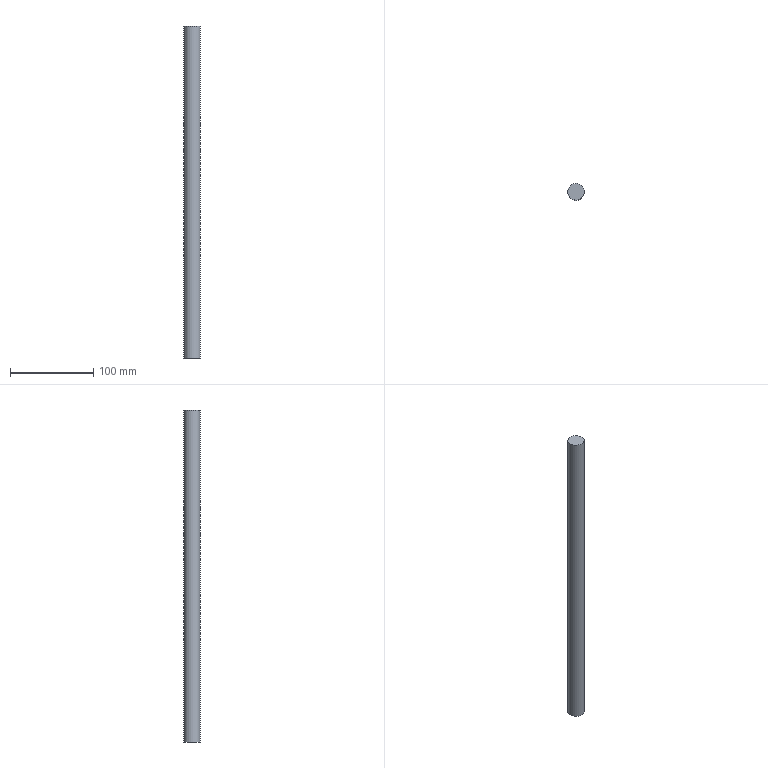Component | NX | D_2 | 1 solid | 3 faces | box 20 x 20 x 400 mm | volume 125664 mm3 | plane 2 | cylinder 1 | commonest cylinder face diameters 20 x1
STEP:
#1=CARTESIAN_POINT('',(0.,0.,0.));
#2=DIRECTION('',(0.,0.,1.));
#3=DIRECTION('',(1.,0.,0.));
#4=AXIS2_PLACEMENT_3D('',#1,#2,#3);
#5=CARTESIAN_POINT('',(850.763,-18.9,-161.891));
#6=VERTEX_POINT('',#5);
#7=CARTESIAN_POINT('',(860.,-15.069,-161.891));
#8=DIRECTION('',(0.,0.,-1.));
#9=DIRECTION('',(-0.9237,-0.383,0.));
#10=AXIS2_PLACEMENT_3D('',#7,#8,#9);
#11=CIRCLE('',#10,10.);
#12=CARTESIAN_POINT('',(860.,-15.069,-161.891));
#13=DIRECTION('',(0.,0.,1.));
#14=DIRECTION('',(0.9237,0.383,0.));
#15=AXIS2_PLACEMENT_3D('',#12,#13,#14);
#16=CYLINDRICAL_SURFACE('',#15,10.);
#17=CARTESIAN_POINT('',(9.425,0.));
#18=DIRECTION('',(-1.,0.));
#19=VECTOR('',#18,1.);
#20=LINE('',#17,#19);
#21=(GEOMETRIC_REPRESENTATION_CONTEXT(2)PARAMETRIC_REPRESENTATION_CONTEXT()REPRESENTATION_CONTEXT('',''));
#22=DEFINITIONAL_REPRESENTATION('',(#20),#21);
#23=PCURVE('',#16,#22);
#24=CARTESIAN_POINT('',(860.,-15.069,-161.891));
#25=DIRECTION('',(0.,0.,-1.));
#26=DIRECTION('',(-0.9237,-0.383,0.));
#27=AXIS2_PLACEMENT_3D('',#24,#25,#26);
#28=PLANE('',#27);
#29=CARTESIAN_POINT('',(0.,0.));
#30=DIRECTION('',(1.,0.));
#31=AXIS2_PLACEMENT_2D('',#29,#30);
#32=CIRCLE('',#31,10.);
#33=(GEOMETRIC_REPRESENTATION_CONTEXT(2)PARAMETRIC_REPRESENTATION_CONTEXT()REPRESENTATION_CONTEXT('',''));
#34=DEFINITIONAL_REPRESENTATION('',(#32),#33);
#35=PCURVE('',#28,#34);
#36=SURFACE_CURVE('',#11,(#23,#35),.PCURVE_S1.);
#37=EDGE_CURVE('',#6,#6,#36,.T.);
#38=ORIENTED_EDGE('',*,*,#37,.F.);
#39=CARTESIAN_POINT('',(850.763,-18.9,238.109));
#40=VERTEX_POINT('',#39);
#41=CARTESIAN_POINT('',(850.763,-18.9,-161.891));
#42=CARTESIAN_POINT('',(850.763,-18.9,238.109));
#43=B_SPLINE_CURVE_WITH_KNOTS('',1,(#41,#42),.UNSPECIFIED.,.F.,.F.,(2,2),(0.,400.),.PIECEWISE_BEZIER_KNOTS.);
#44=CARTESIAN_POINT('',(9.425,0.));
#45=DIRECTION('',(0.,1.));
#46=VECTOR('',#45,1.);
#47=LINE('',#44,#46);
#48=(GEOMETRIC_REPRESENTATION_CONTEXT(2)PARAMETRIC_REPRESENTATION_CONTEXT()REPRESENTATION_CONTEXT('',''));
#49=DEFINITIONAL_REPRESENTATION('',(#47),#48);
#50=PCURVE('',#16,#49);
#51=CARTESIAN_POINT('',(3.142,0.));
#52=DIRECTION('',(0.,1.));
#53=VECTOR('',#52,1.);
#54=LINE('',#51,#53);
#55=(GEOMETRIC_REPRESENTATION_CONTEXT(2)PARAMETRIC_REPRESENTATION_CONTEXT()REPRESENTATION_CONTEXT('',''));
#56=DEFINITIONAL_REPRESENTATION('',(#54),#55);
#57=PCURVE('',#16,#56);
#58=SEAM_CURVE('',#43,(#50,#57),.PCURVE_S1.);
#59=EDGE_CURVE('',#6,#40,#58,.T.);
#60=ORIENTED_EDGE('',*,*,#59,.T.);
#61=CARTESIAN_POINT('',(860.,-15.069,238.109));
#62=DIRECTION('',(0.,0.,-1.));
#63=DIRECTION('',(-0.9237,-0.383,0.));
#64=AXIS2_PLACEMENT_3D('',#61,#62,#63);
#65=CIRCLE('',#64,10.);
#66=CARTESIAN_POINT('',(9.425,400.));
#67=DIRECTION('',(-1.,0.));
#68=VECTOR('',#67,1.);
#69=LINE('',#66,#68);
#70=(GEOMETRIC_REPRESENTATION_CONTEXT(2)PARAMETRIC_REPRESENTATION_CONTEXT()REPRESENTATION_CONTEXT('',''));
#71=DEFINITIONAL_REPRESENTATION('',(#69),#70);
#72=PCURVE('',#16,#71);
#73=CARTESIAN_POINT('',(860.,-15.069,238.109));
#74=DIRECTION('',(0.,0.,-1.));
#75=DIRECTION('',(-0.9237,-0.383,0.));
#76=AXIS2_PLACEMENT_3D('',#73,#74,#75);
#77=PLANE('',#76);
#78=CARTESIAN_POINT('',(0.,0.));
#79=DIRECTION('',(1.,0.));
#80=AXIS2_PLACEMENT_2D('',#78,#79);
#81=CIRCLE('',#80,10.);
#82=(GEOMETRIC_REPRESENTATION_CONTEXT(2)PARAMETRIC_REPRESENTATION_CONTEXT()REPRESENTATION_CONTEXT('',''));
#83=DEFINITIONAL_REPRESENTATION('',(#81),#82);
#84=PCURVE('',#77,#83);
#85=SURFACE_CURVE('',#65,(#72,#84),.PCURVE_S1.);
#86=EDGE_CURVE('',#40,#40,#85,.T.);
#87=ORIENTED_EDGE('',*,*,#86,.T.);
#88=ORIENTED_EDGE('',*,*,#59,.F.);
#89=EDGE_LOOP('',(#38,#60,#87,#88));
#90=FACE_BOUND('',#89,.T.);
#91=ADVANCED_FACE('',(#90),#16,.T.);
#92=ORIENTED_EDGE('',*,*,#37,.T.);
#93=EDGE_LOOP('',(#92));
#94=FACE_BOUND('',#93,.T.);
#95=ADVANCED_FACE('',(#94),#28,.T.);
#96=ORIENTED_EDGE('',*,*,#86,.F.);
#97=EDGE_LOOP('',(#96));
#98=FACE_BOUND('',#97,.T.);
#99=ADVANCED_FACE('',(#98),#77,.F.);
#100=CLOSED_SHELL('',(#91,#95,#99));
#101=MANIFOLD_SOLID_BREP('',#100);
#102=(LENGTH_UNIT()NAMED_UNIT(*)SI_UNIT(.MILLI.,.METRE.));
#103=UNCERTAINTY_MEASURE_WITH_UNIT(LENGTH_MEASURE(0.00001),#102,'','');
#104=(NAMED_UNIT(*)PLANE_ANGLE_UNIT()SI_UNIT($,.RADIAN.));
#105=(NAMED_UNIT(*)SI_UNIT($,.STERADIAN.)SOLID_ANGLE_UNIT());
#106=(GEOMETRIC_REPRESENTATION_CONTEXT(3)GLOBAL_UNCERTAINTY_ASSIGNED_CONTEXT((#103))GLOBAL_UNIT_ASSIGNED_CONTEXT((#102,#104,#105))REPRESENTATION_CONTEXT('',''));
#107=ADVANCED_BREP_SHAPE_REPRESENTATION('',(#4,#101),#106);